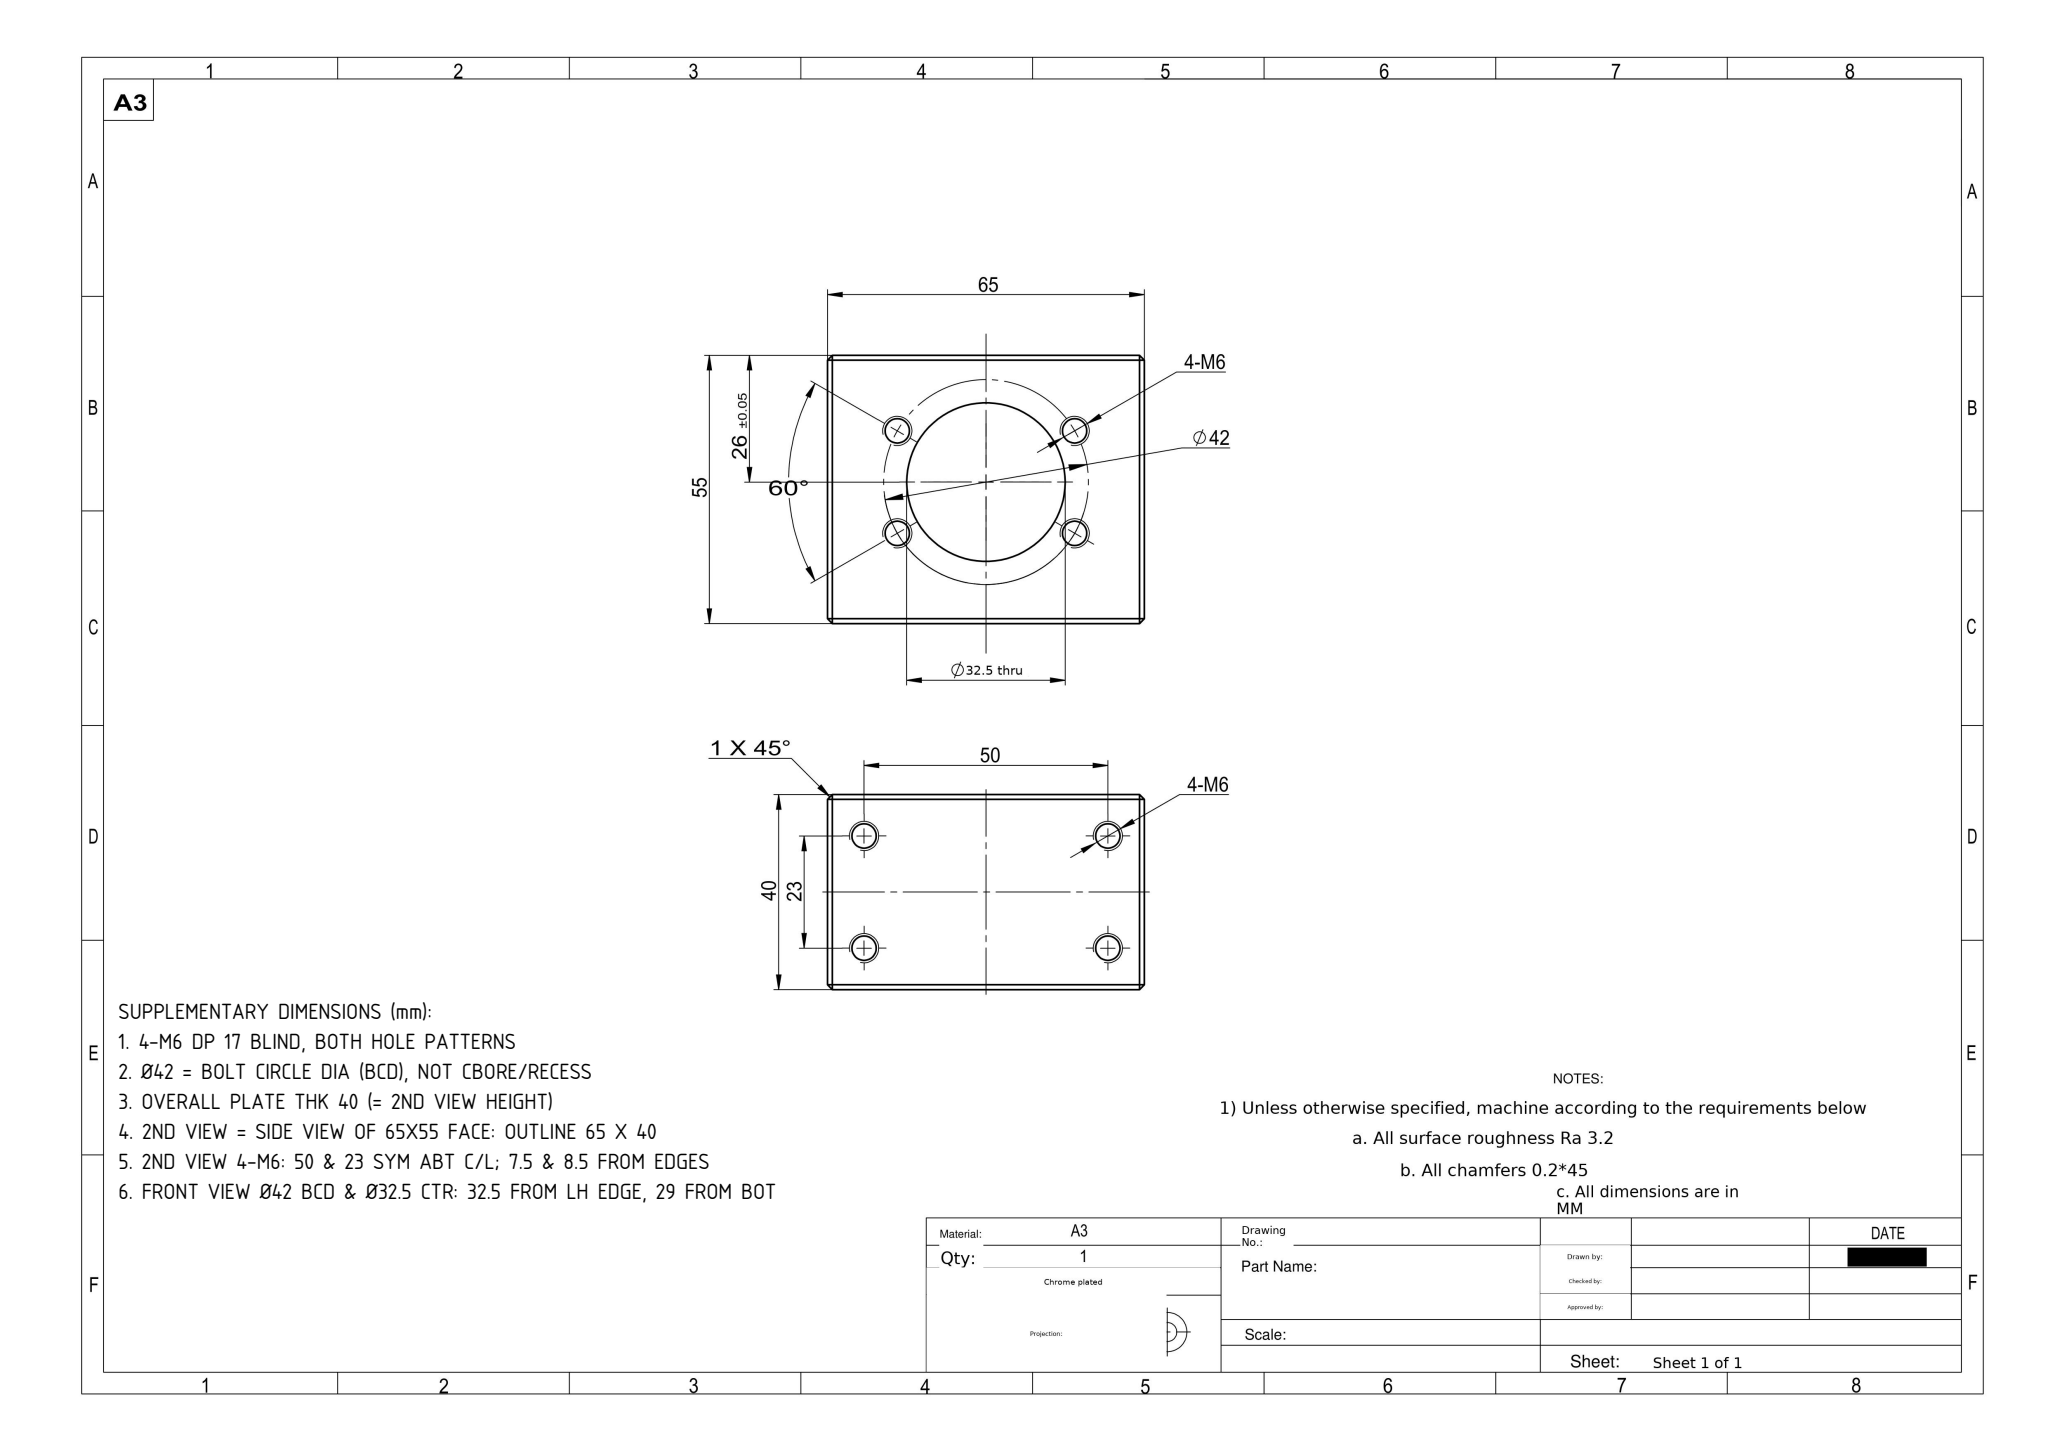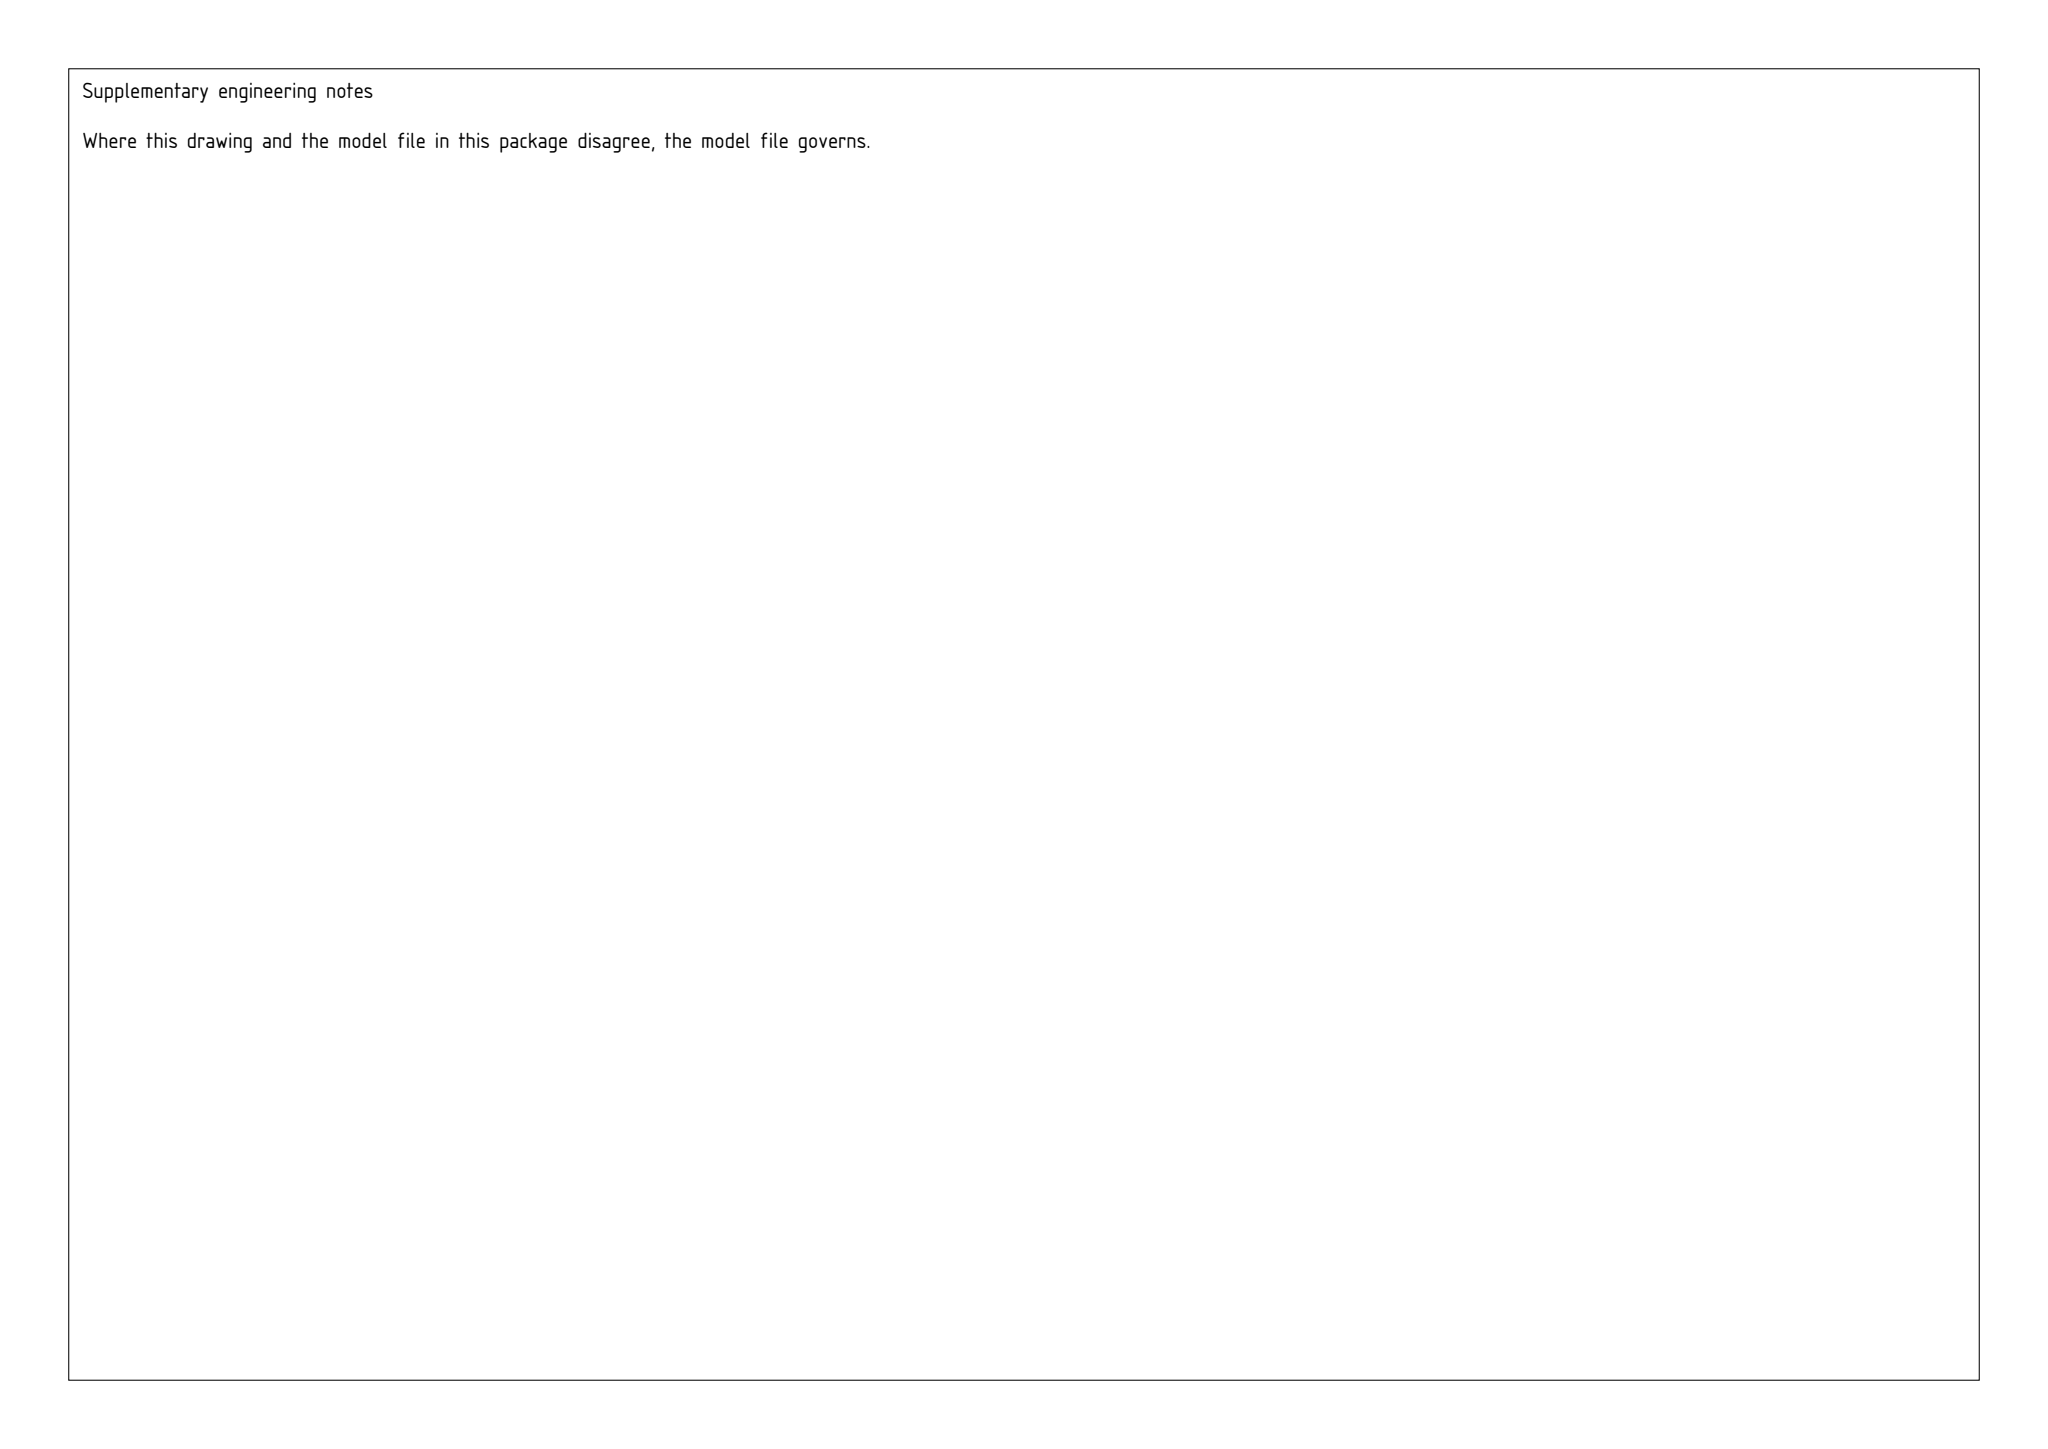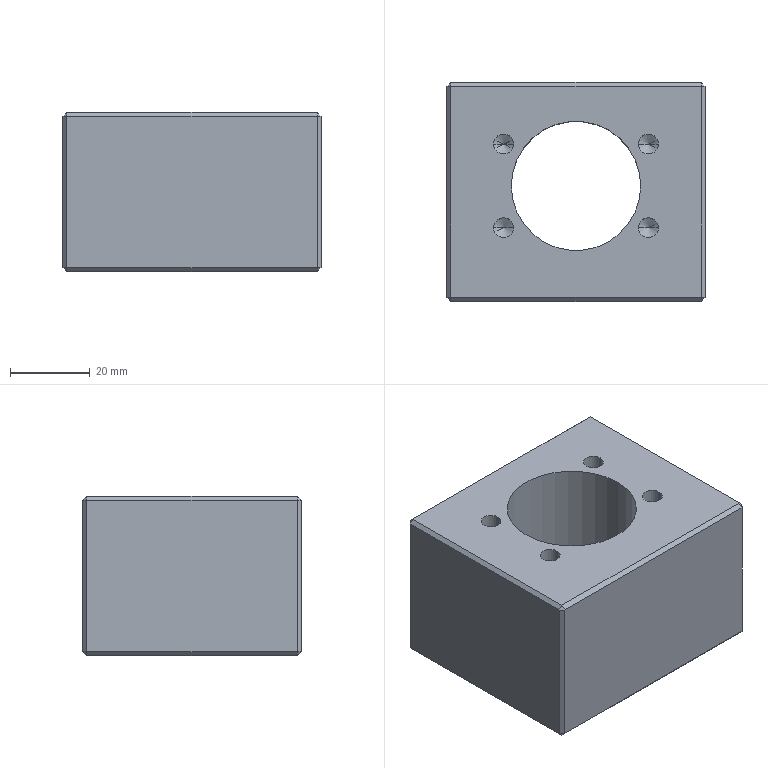Part | SolidWorks | mm | 1 solid | 60 faces | box 65 x 55 x 40 mm | volume 106753 mm3 | plane 26 | cylinder 18 | cone 16 | commonest cylinder face diameters 5 x16 32.5 x2
build123d program:
from build123d import *

# Parameters (mm, degrees)
SKETCH1_W             = 65
SKETCH1_H             = 55
SKETCH1_R             = 16.25
BOSS_EXTRUDE1_DEPTH   = 20
M6_TAPPED_HOLE1_D     = 5
M6_TAPPED_HOLE1_DEPTH = 17
M6_TAPPED_HOLE1_TIP   = 1.502
M6_TAPPED_HOLE2_D     = 5
M6_TAPPED_HOLE2_DEPTH = 17
M6_TAPPED_HOLE2_TIP   = 1.502
CHAMFER1_SIZE         = 1


with BuildPart() as part:
    # Sketch1 → Boss-Extrude1 (new, symmetric)
    with BuildSketch(Plane.XY):
        Rectangle(SKETCH1_W, SKETCH1_H)
        with Locations((0, 1.5)):
            Circle(SKETCH1_R, mode=Mode.SUBTRACT)
    extrude(amount=BOSS_EXTRUDE1_DEPTH, both=True)

    # M6 Tapped Hole1
    with Locations(Plane.XY.offset(20)):
        with Locations((-18.187, 12), (18.187, 12), (-18.187, -9), (18.187, -9)):
            Hole(M6_TAPPED_HOLE1_D / 2, depth=M6_TAPPED_HOLE1_DEPTH)
            with Locations((0, 0, -(M6_TAPPED_HOLE1_DEPTH + M6_TAPPED_HOLE1_TIP / 2))):  # 118° drill point
                Cone(0, M6_TAPPED_HOLE1_D / 2, M6_TAPPED_HOLE1_TIP, mode=Mode.SUBTRACT)

    # M6 Tapped Hole2
    with Locations(Plane(origin=(0, 27.5, 0), x_dir=(1, 0, 0), z_dir=(0, 1, 0))):
        with Locations((-25, 11.5), (-25, -11.5), (25, -11.5), (25, 11.5)):
            Hole(M6_TAPPED_HOLE2_D / 2, depth=M6_TAPPED_HOLE2_DEPTH)
            with Locations((0, 0, -(M6_TAPPED_HOLE2_DEPTH + M6_TAPPED_HOLE2_TIP / 2))):  # 118° drill point
                Cone(0, M6_TAPPED_HOLE2_D / 2, M6_TAPPED_HOLE2_TIP, mode=Mode.SUBTRACT)

    # Chamfer1
    chamfer1_edges = [part.edges().sort_by_distance(p)[0] for p in [
        (-32.5, 0, 20),
        (0, -27.5, 20),
        (32.5, 0, 20),
        (0, -27.5, -20),
        (-32.5, 0, -20),
        (0, 27.5, -20),
        (32.5, 0, -20),
        (0, 27.5, 20),
        (32.5, -27.5, 0),
        (-32.5, -27.5, 0),
        (-32.5, 27.5, 0),
        (32.5, 27.5, 0),
    ]]
    chamfer(chamfer1_edges, length=CHAMFER1_SIZE)


solid = part.part